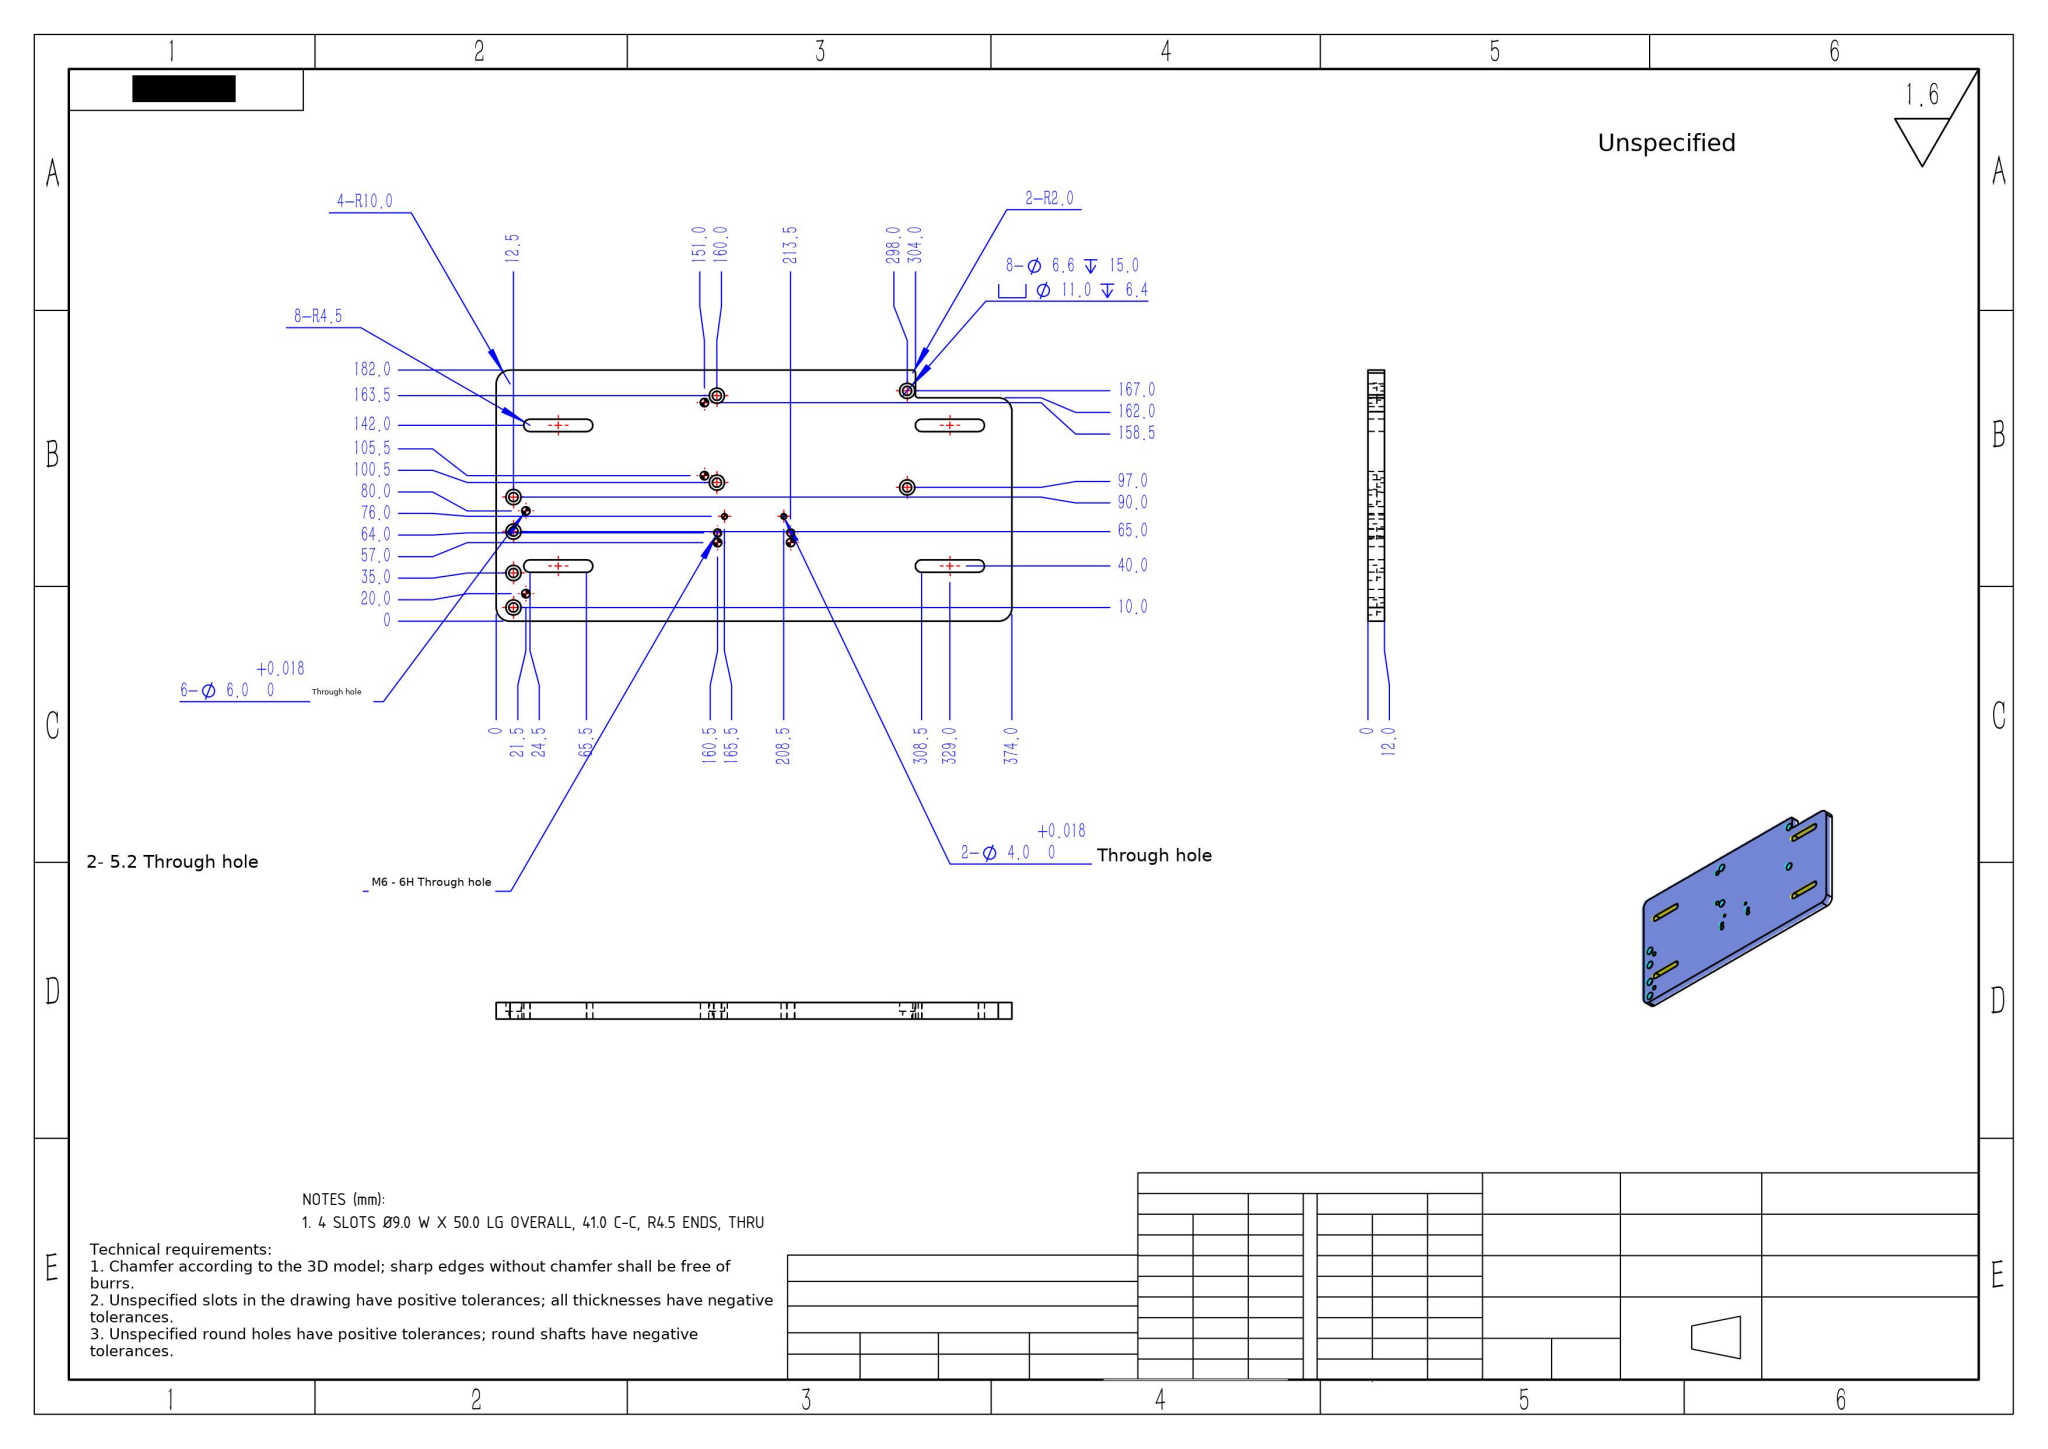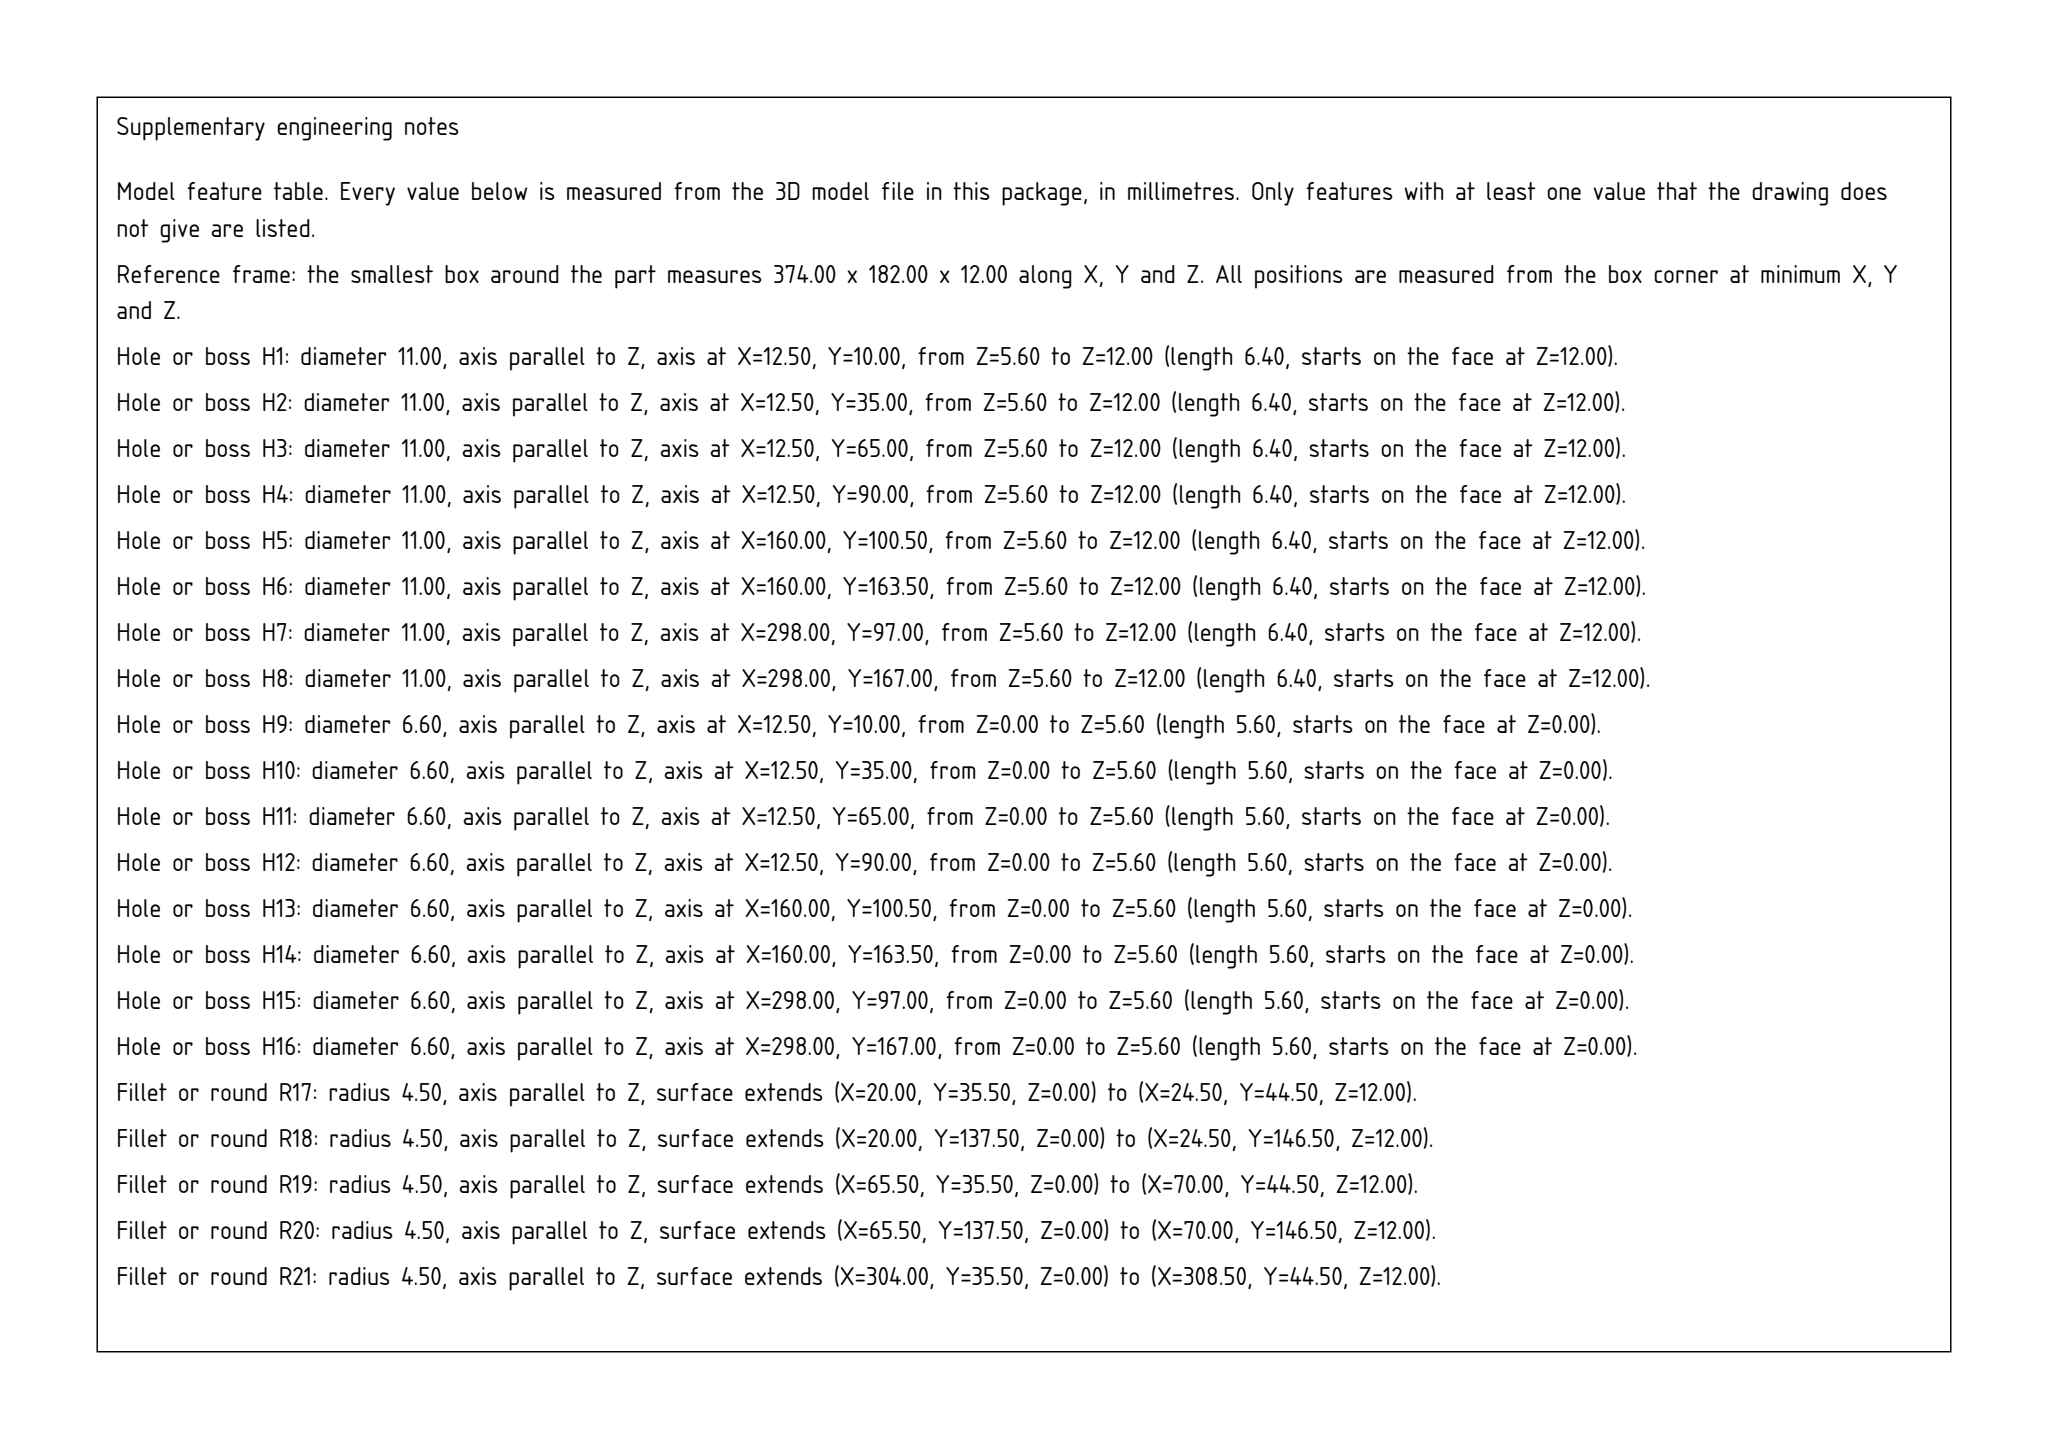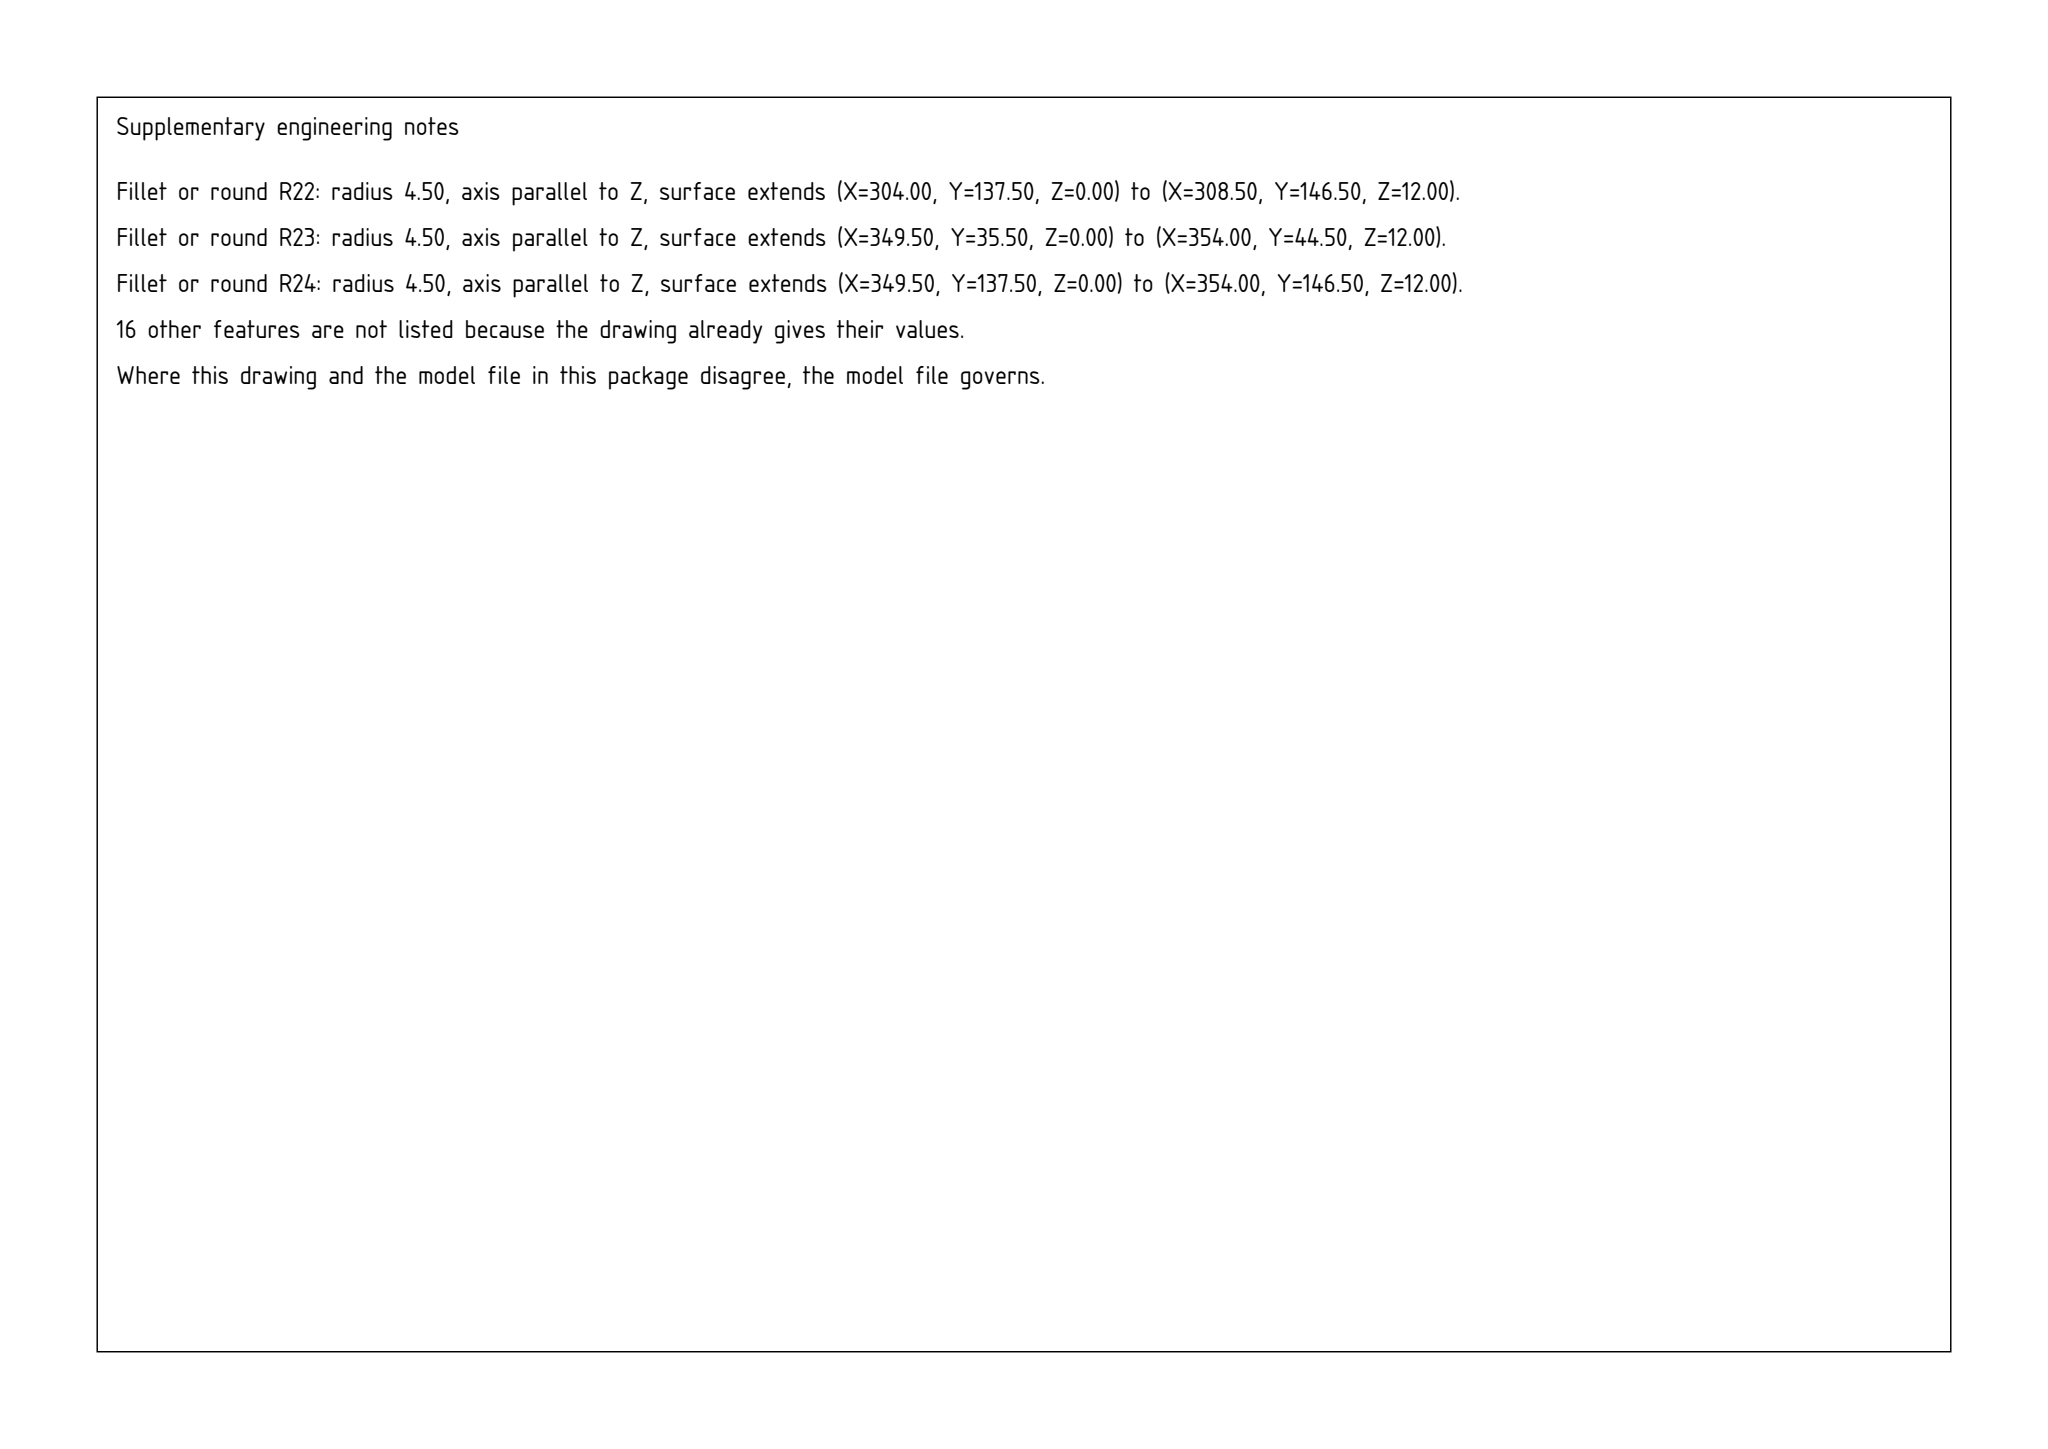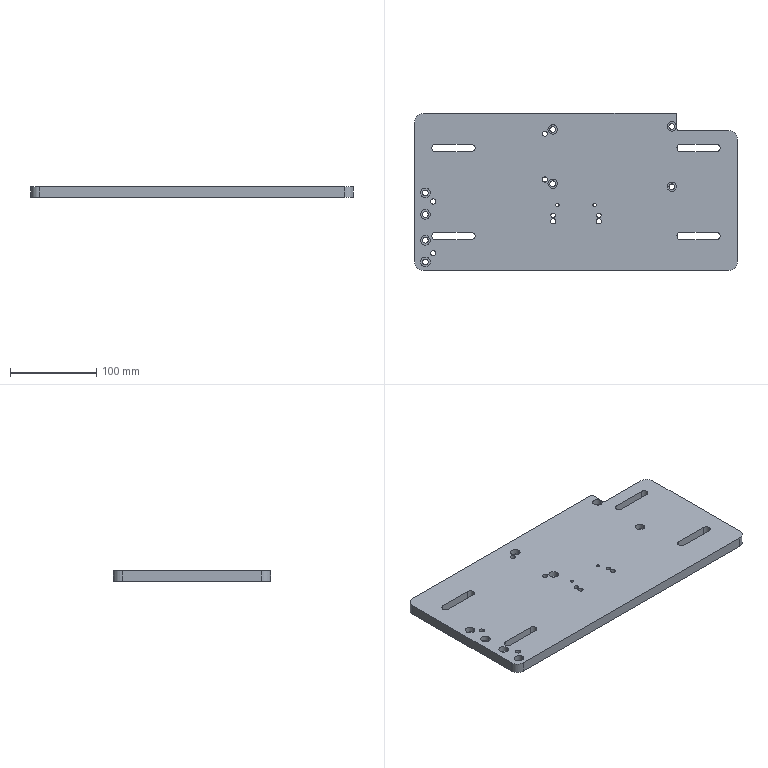Part | SolidWorks | mm | 1 solid | 94 faces | box 374 x 182 x 12 mm | volume 768975 mm3 | cylinder 70 | plane 24 | commonest cylinder face diameters 11 x16 6.6 x16 6 x12 9 x12 4 x6 5.2 x4 20 x4
Drawing notes:
4 SLOTS Ø9.0 W X 50.0 LG OVERALL, 41.0 C-C, R4.5 ENDS, THRU | from the solid: Ø9.0 z-cyls (len 12.0 = full thk) at x=24.5/65.5 and 308.5/349.5, y=40.0 & 142.0: width 9, C-C 41, overall 41+9=50